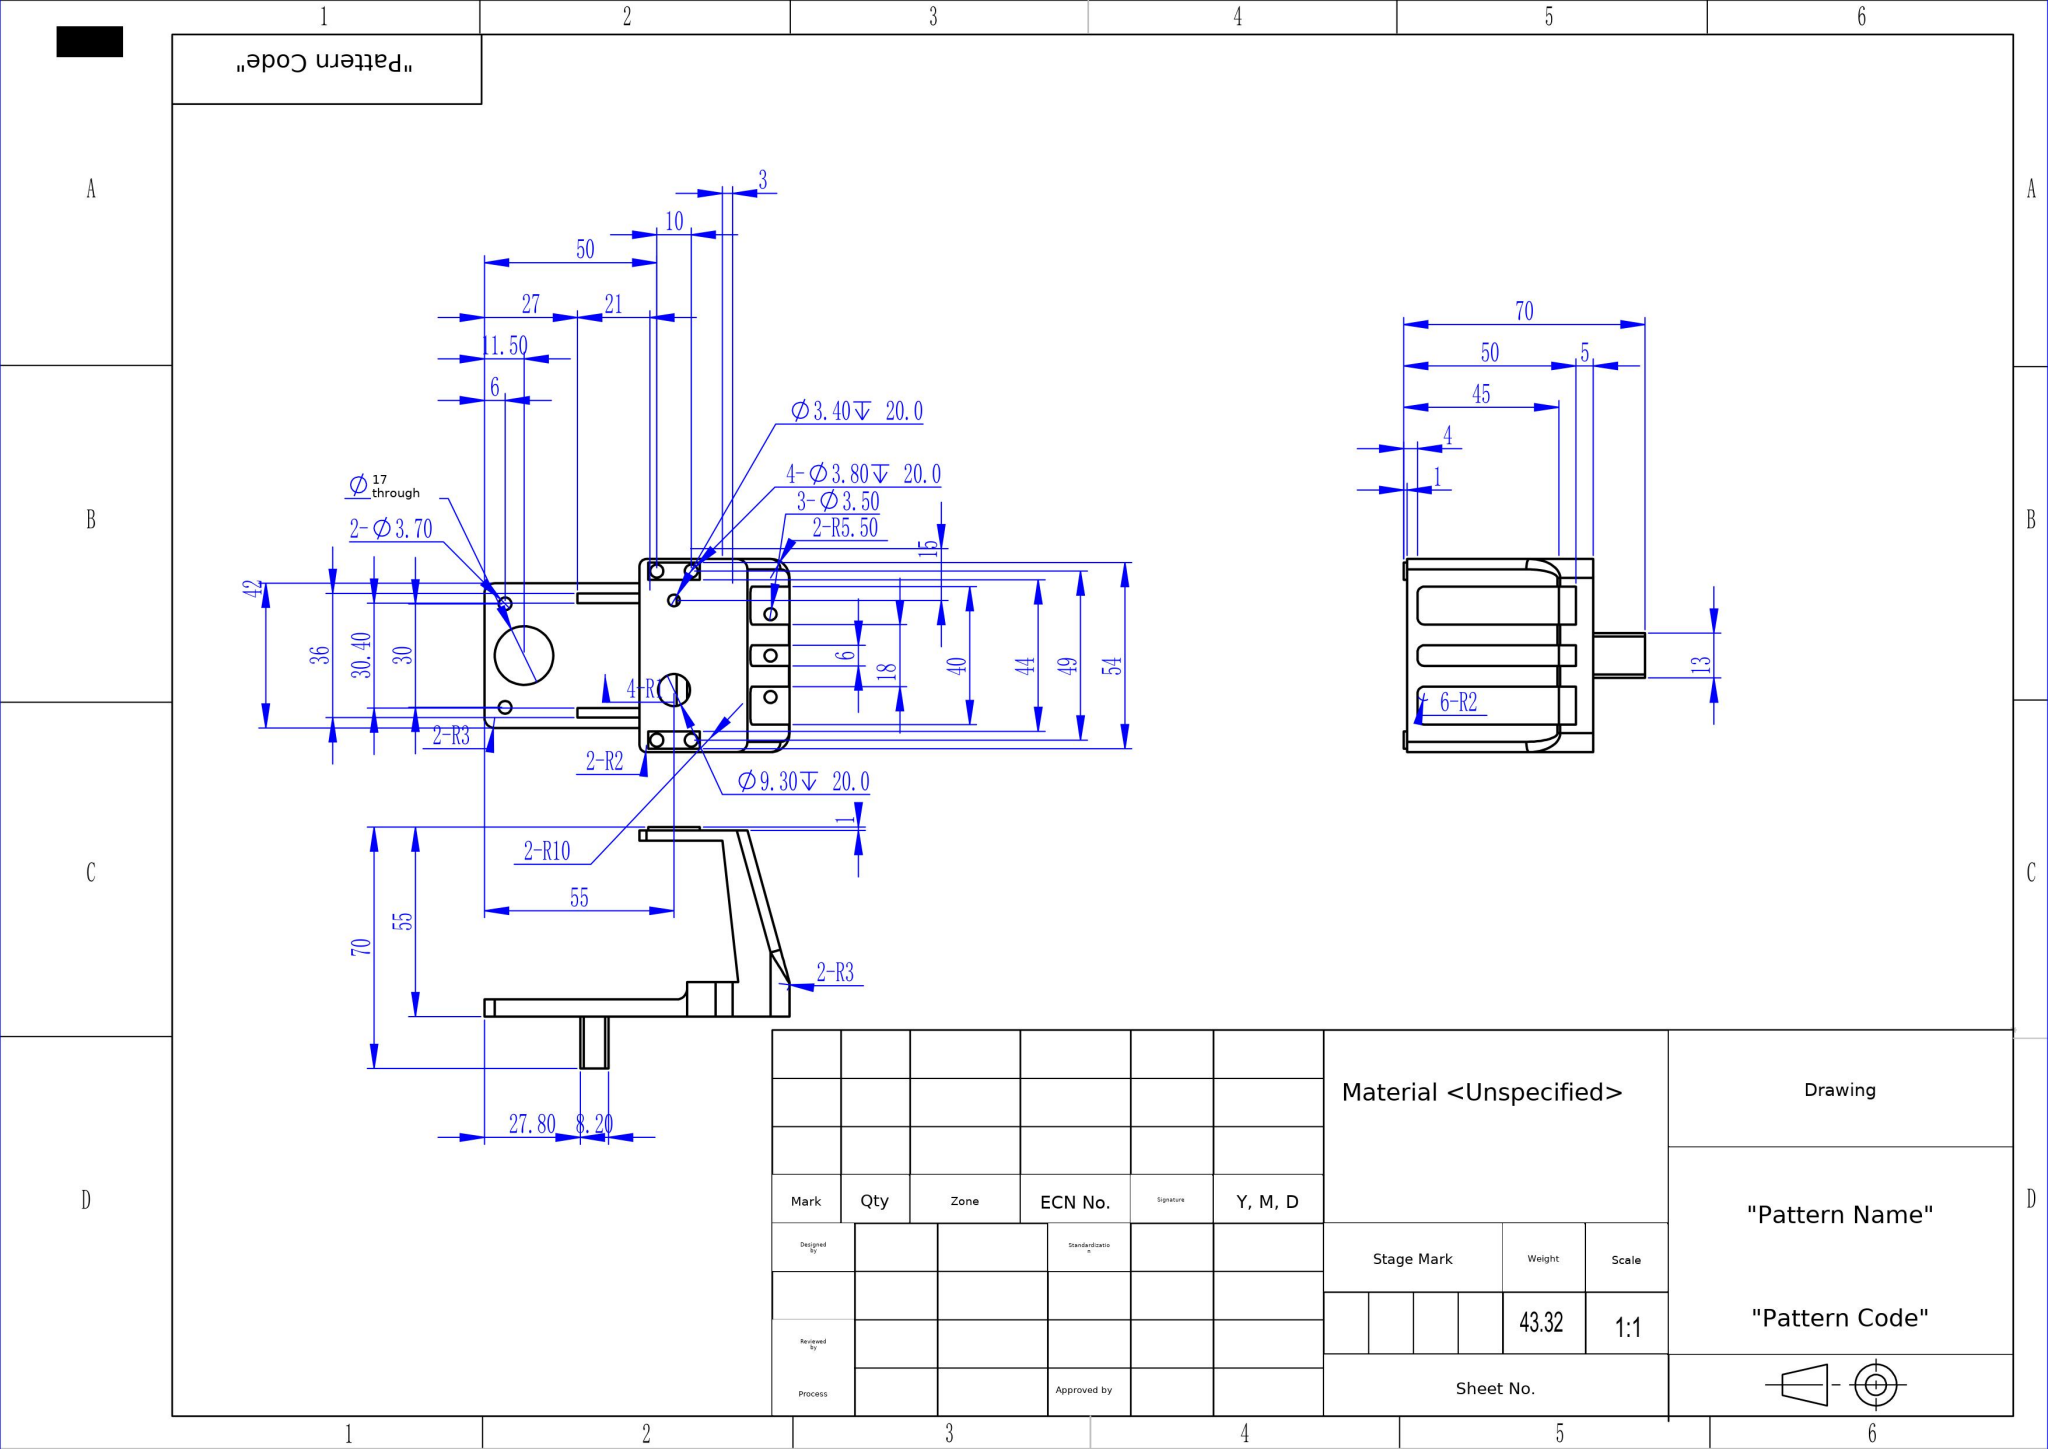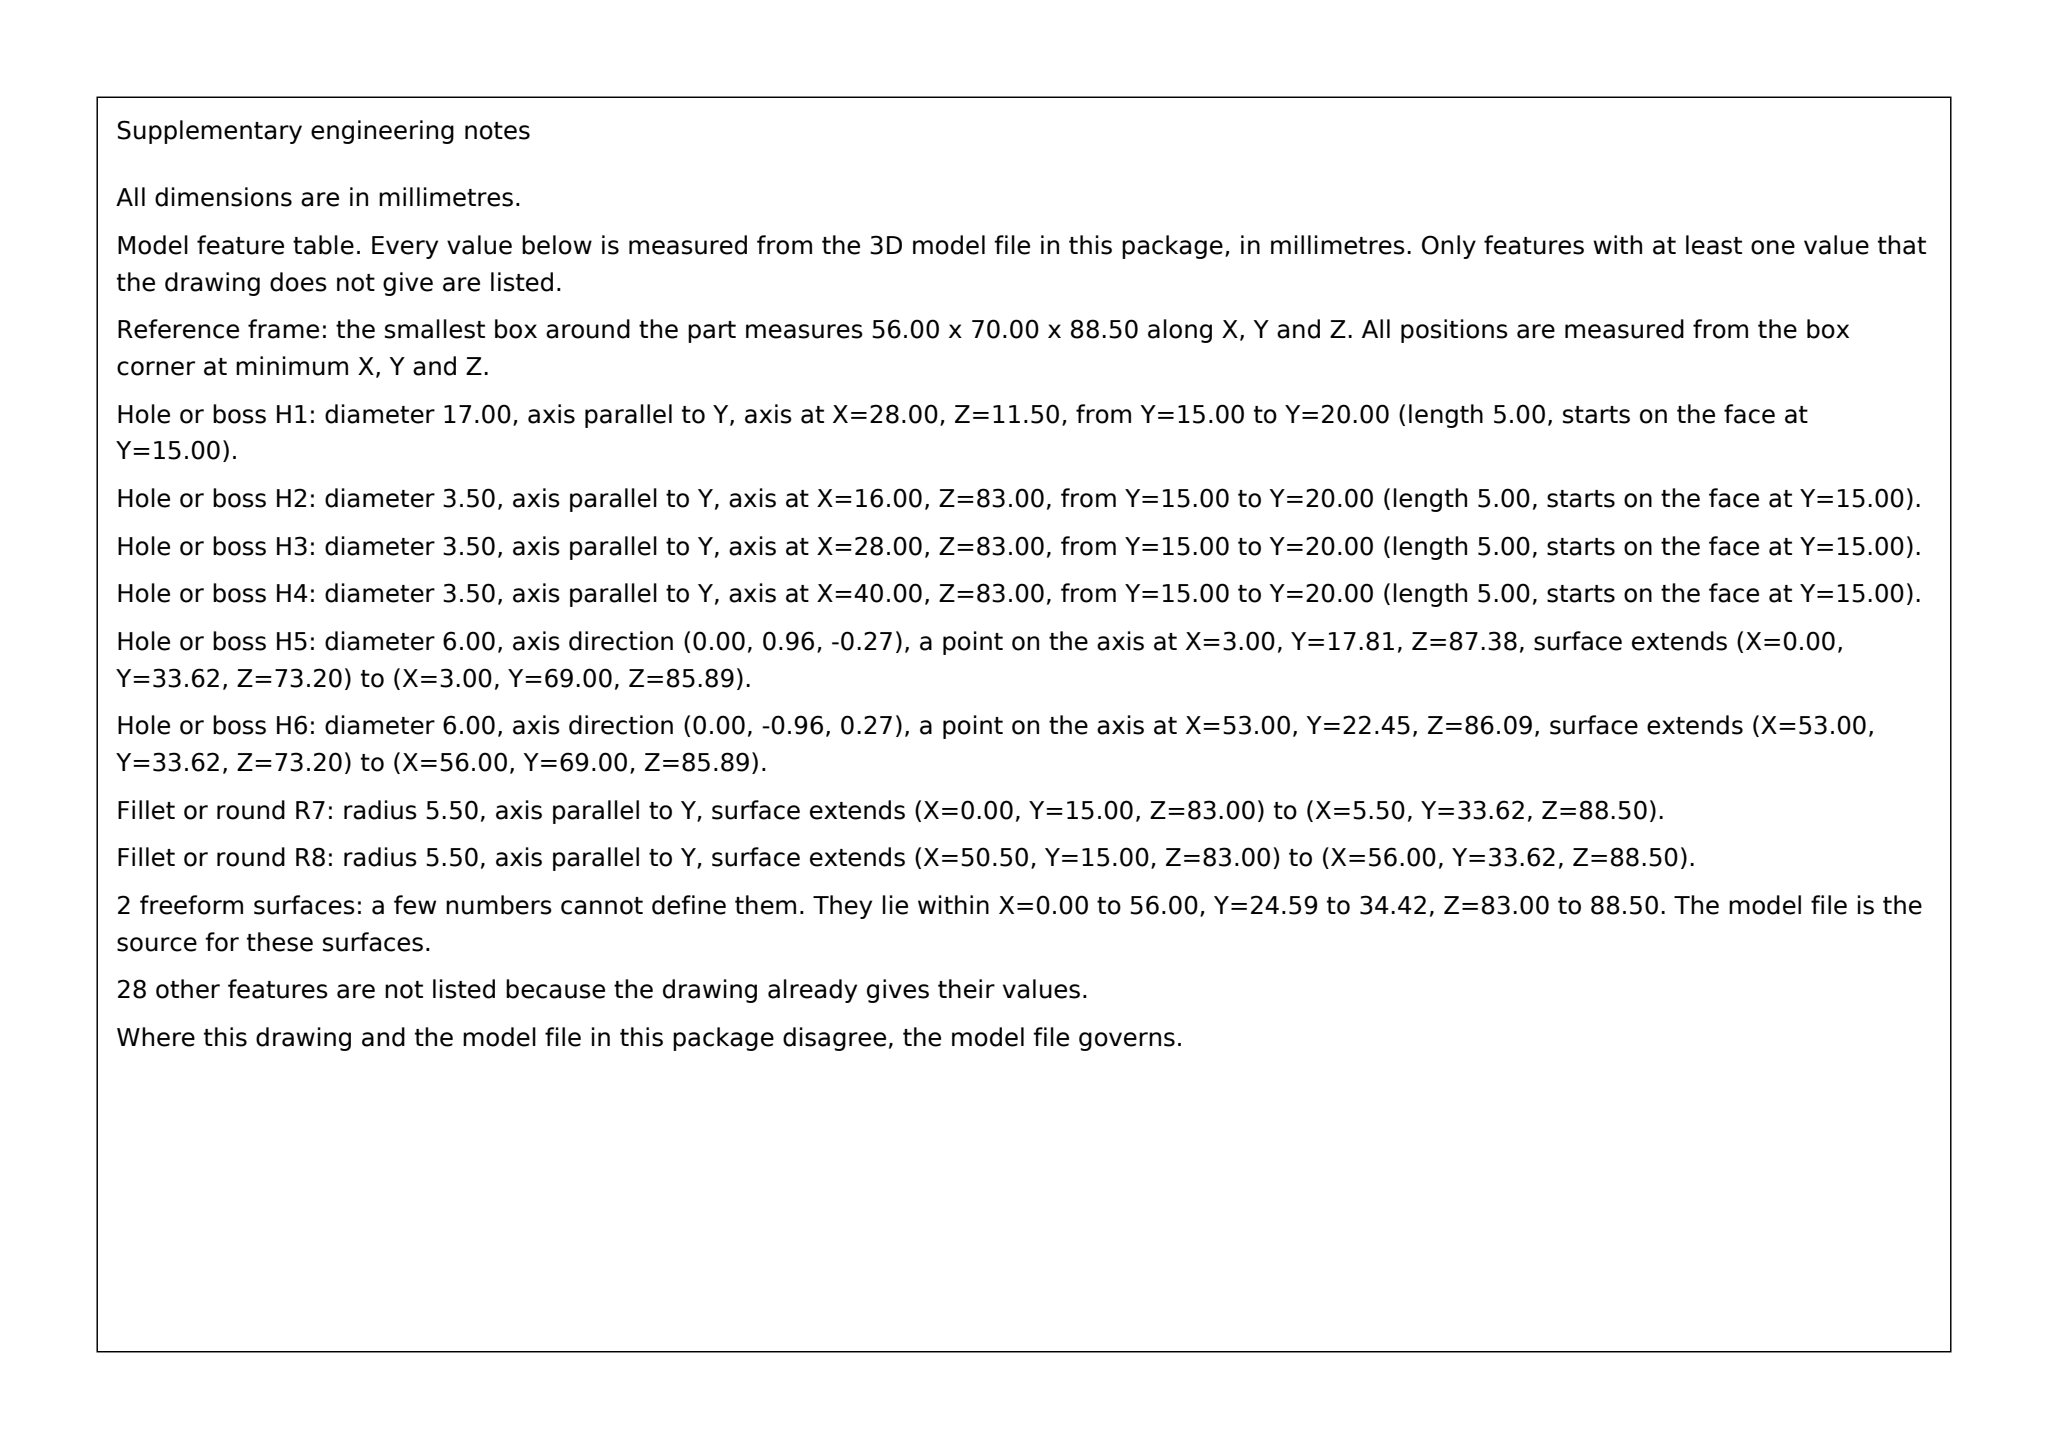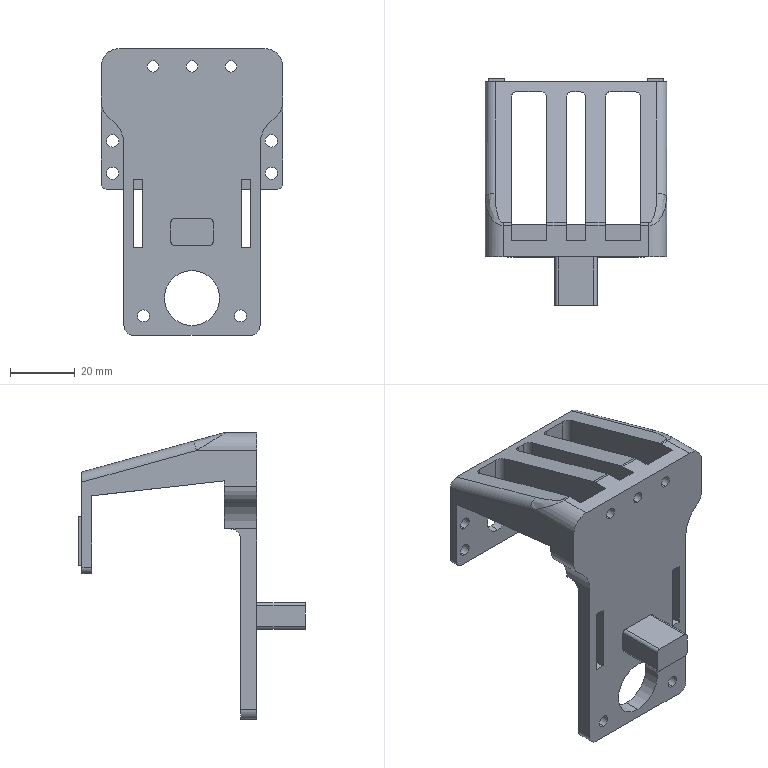Part | SolidWorks | mm | 1 solid | 106 faces | box 56 x 70 x 88.5 mm | volume 43316 mm3 | plane 53 | cylinder 51 | spline 2 | commonest cylinder face diameters 6 x9 3.8 x8 4 x8 3.5 x6 3.7 x4 2 x4 9.3 x2 3.4 x2